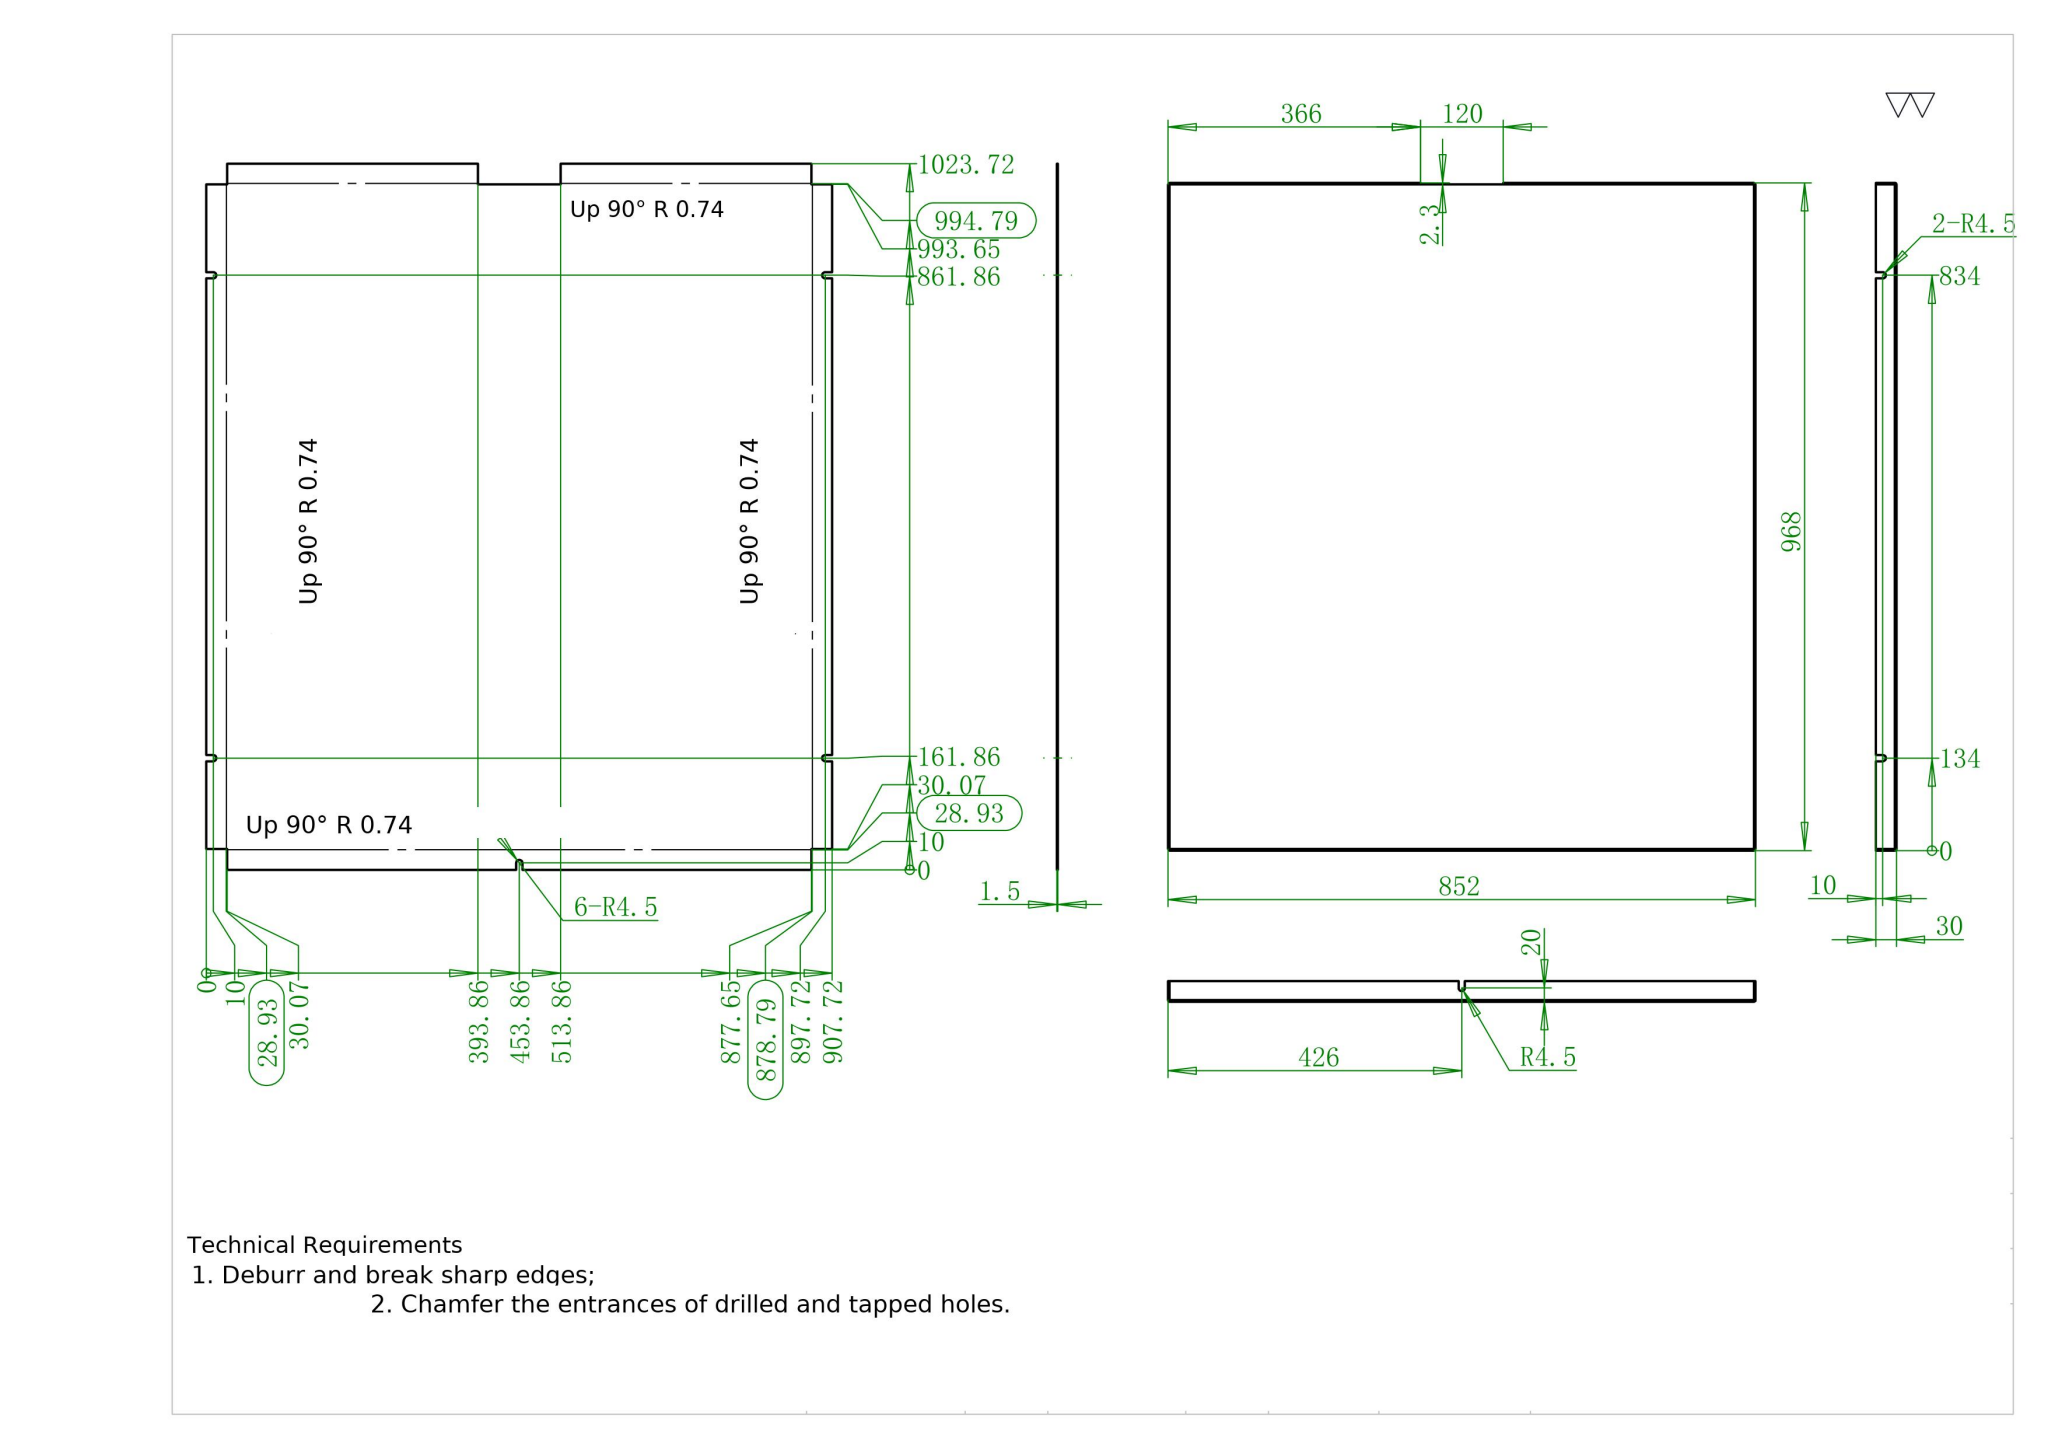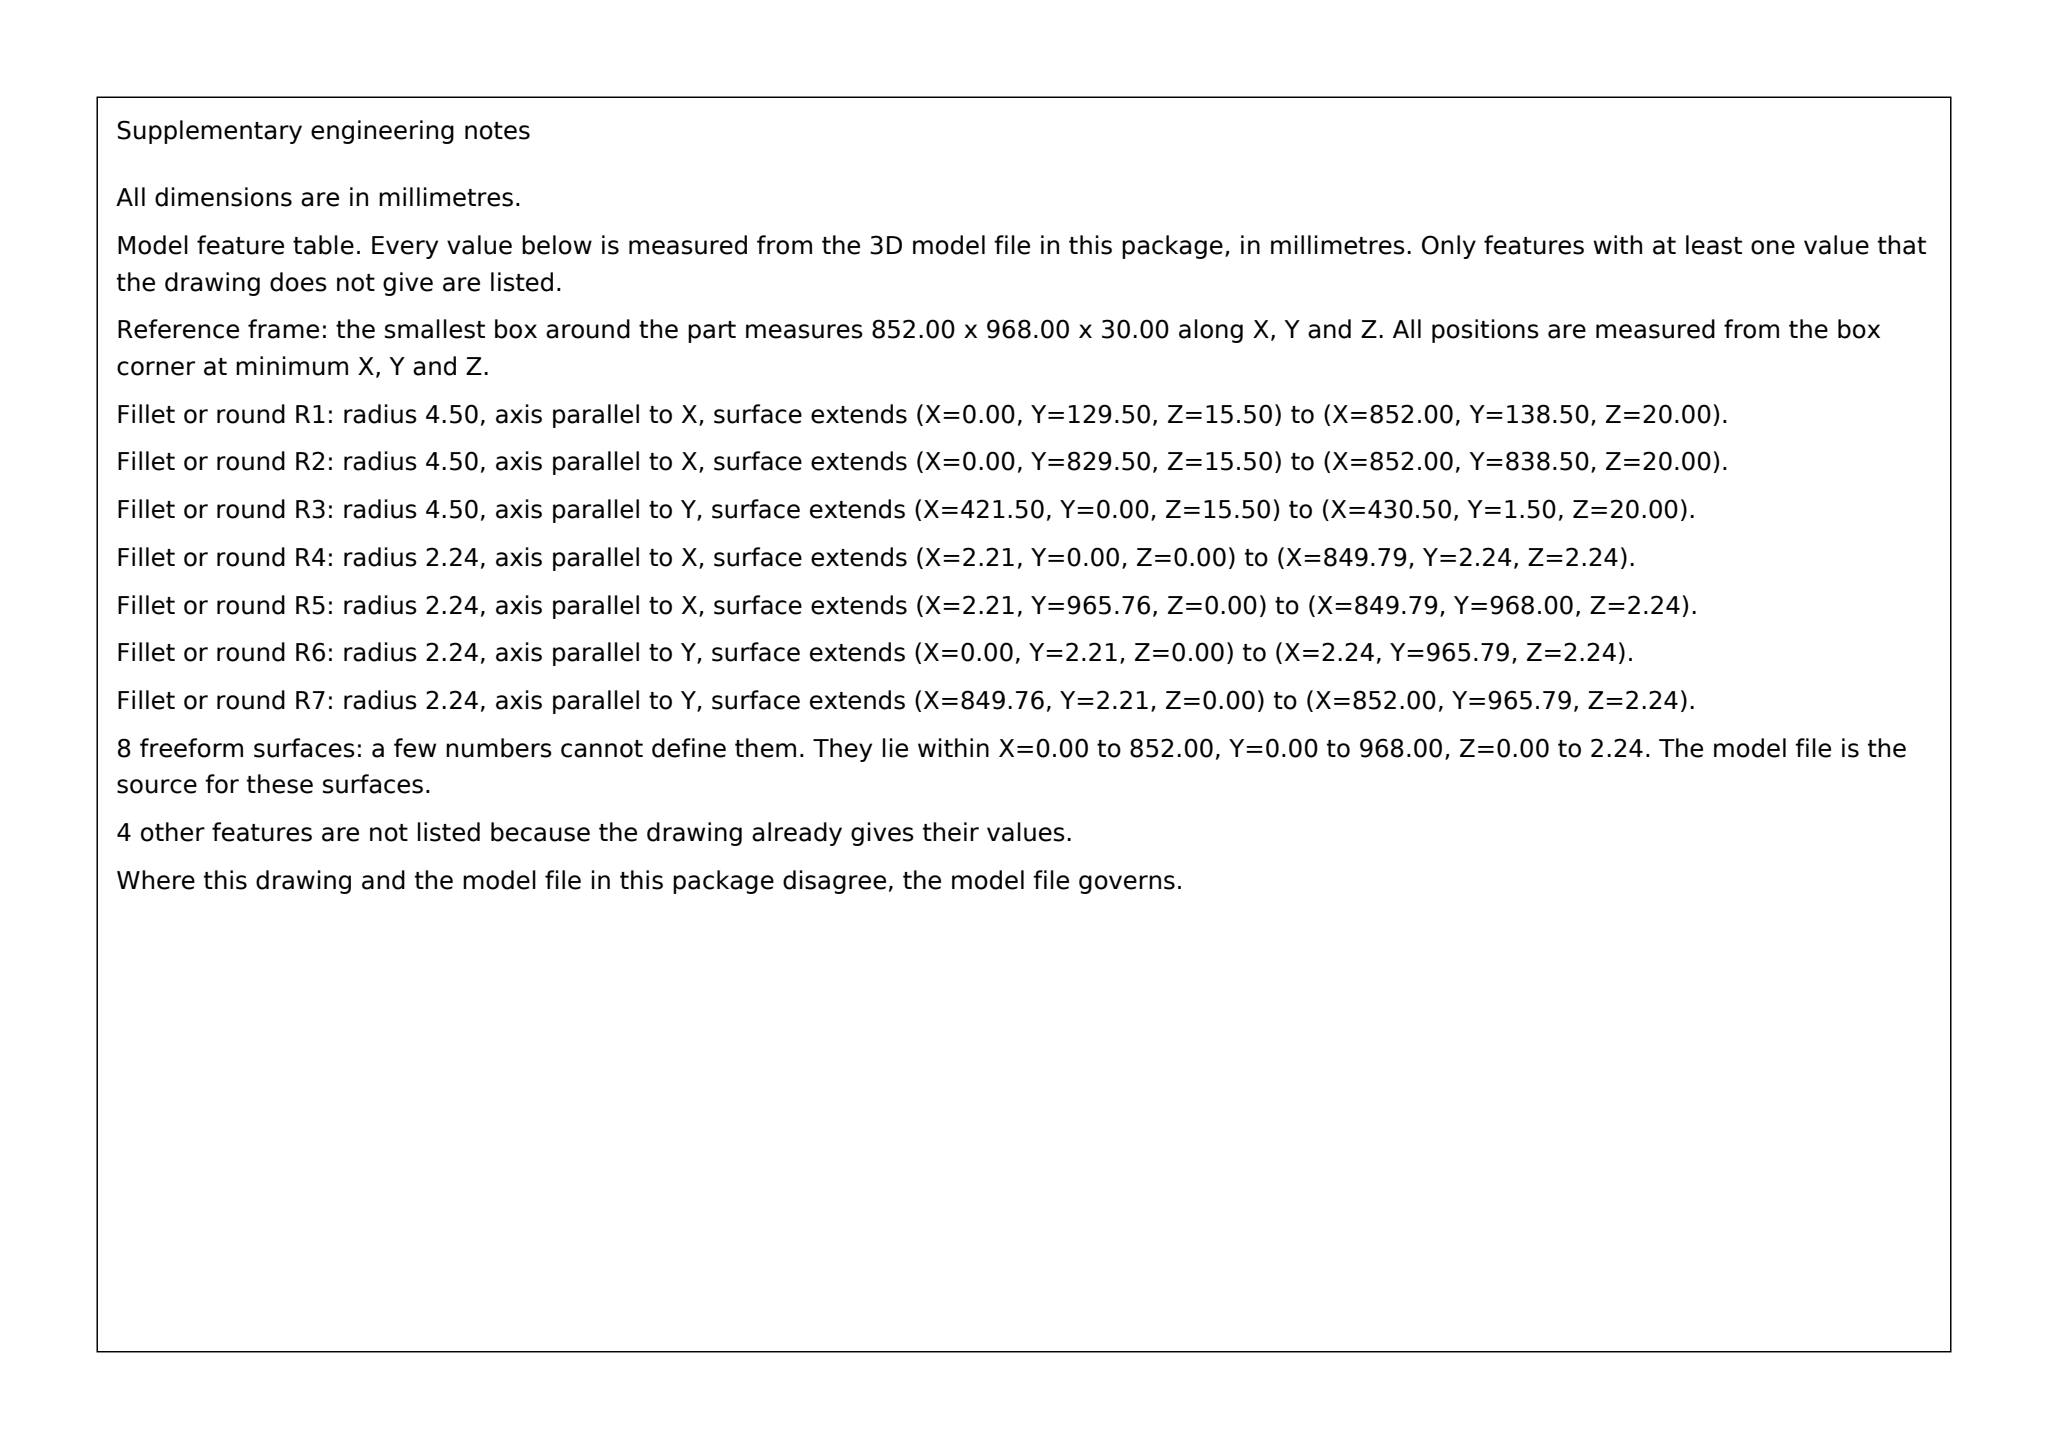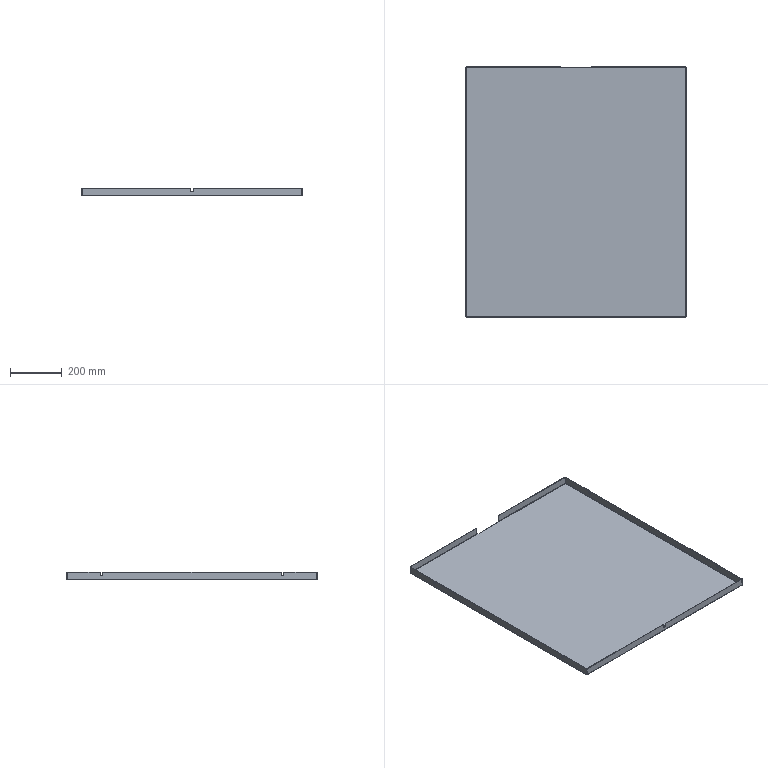Part | SolidWorks | mm | 1 solid | 67 faces | box 852 x 968 x 30 mm | volume 1382132 mm3 | plane 44 | cylinder 15 | spline 8 | commonest cylinder face diameters 4.473 x5 1.473 x5 9 x5